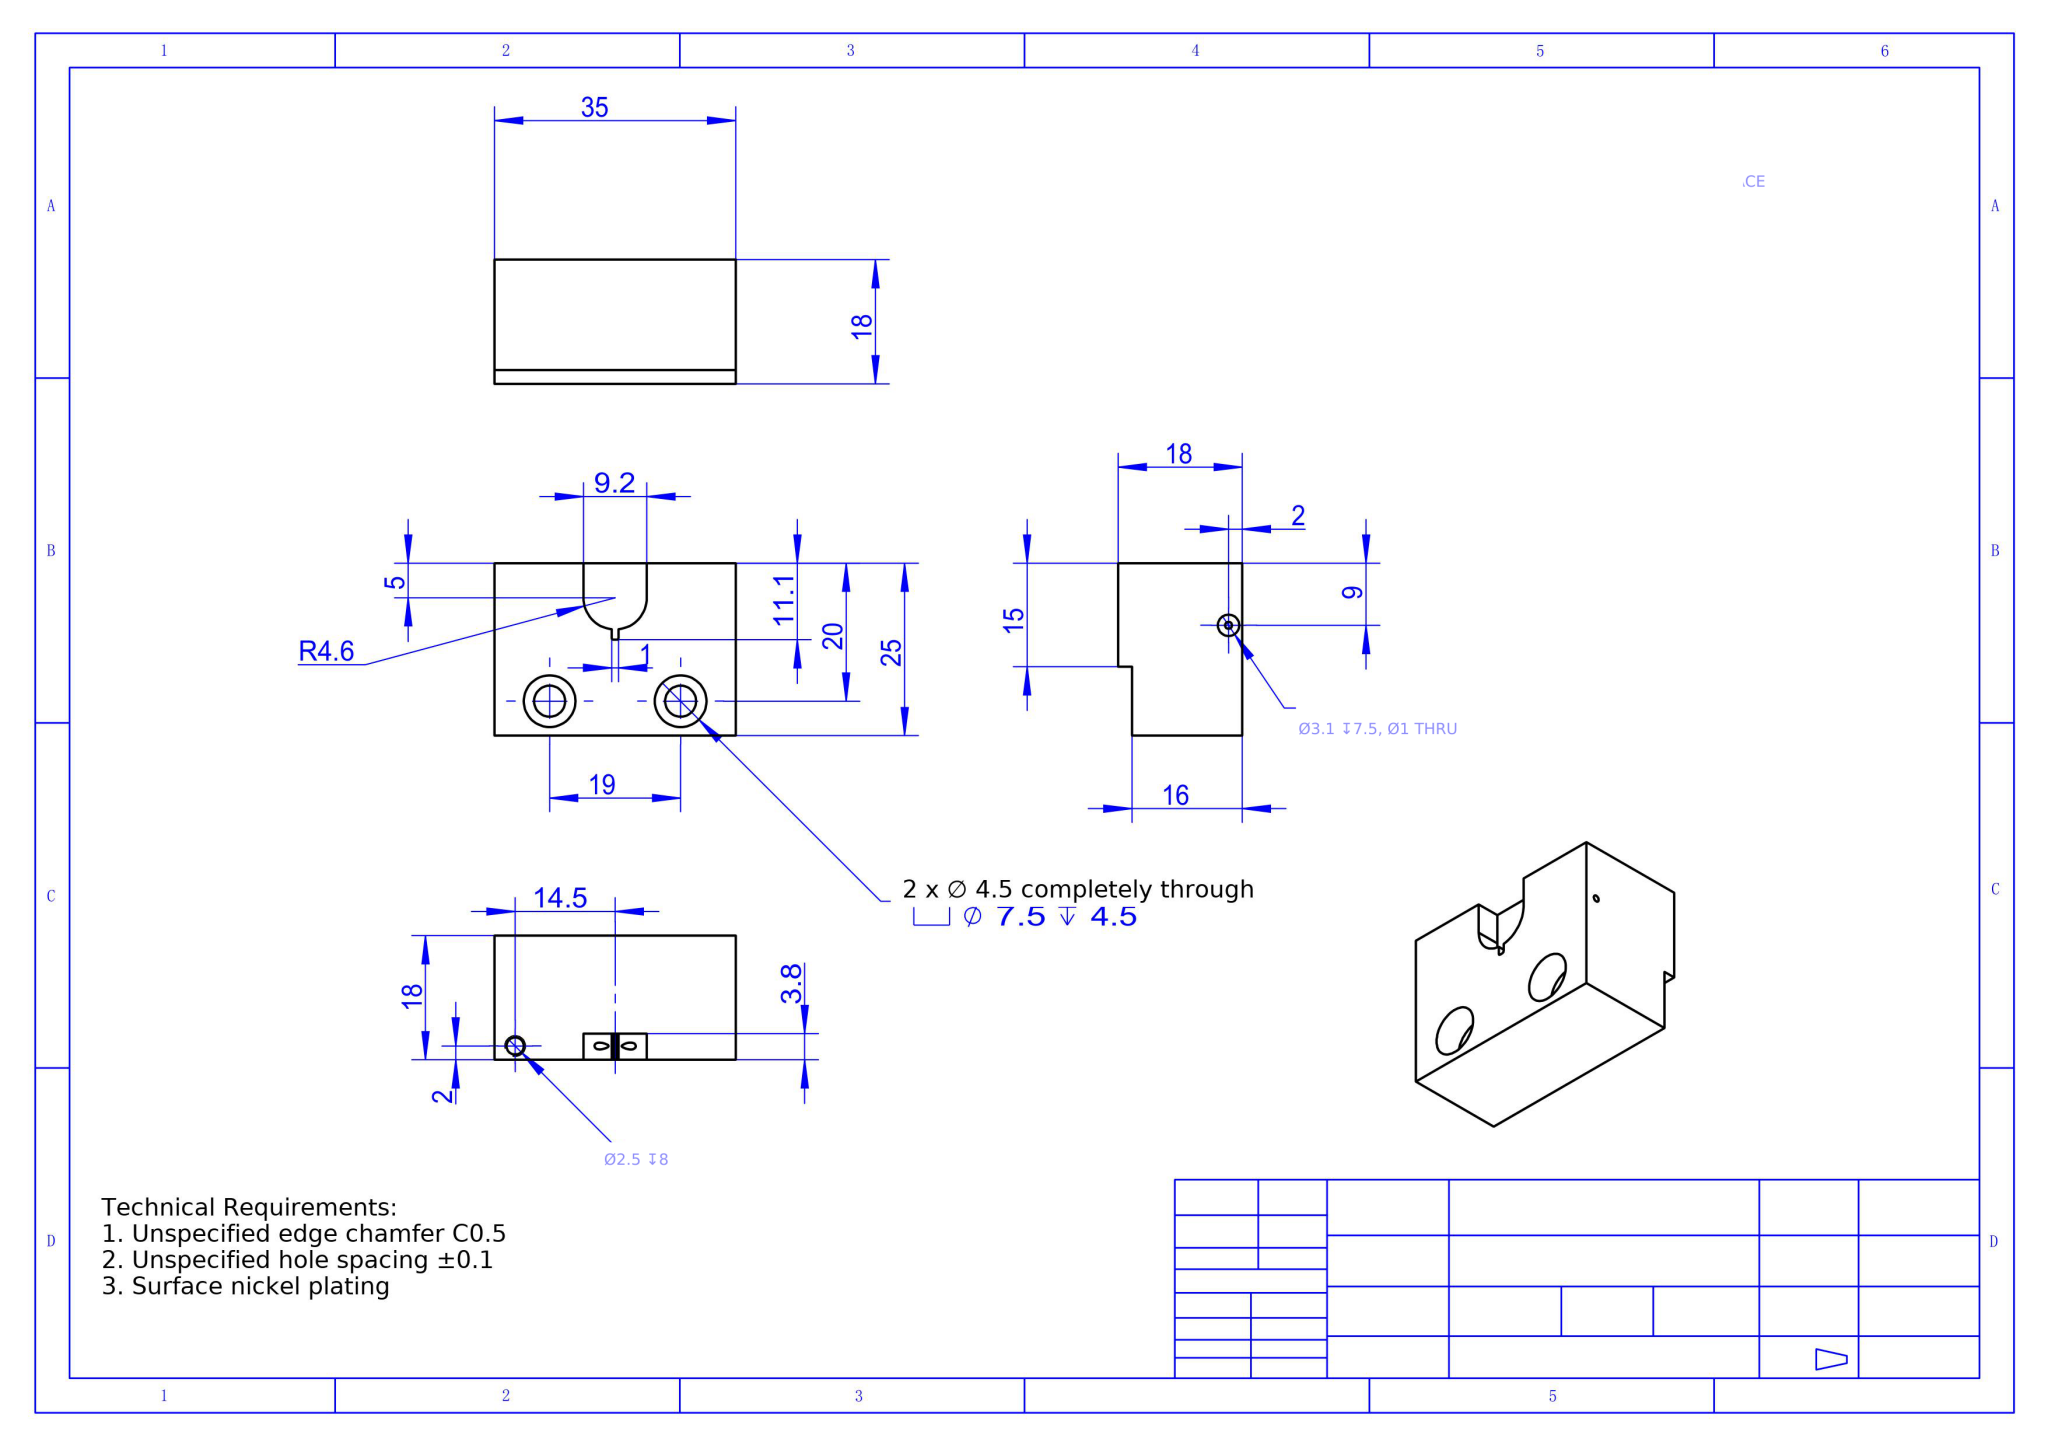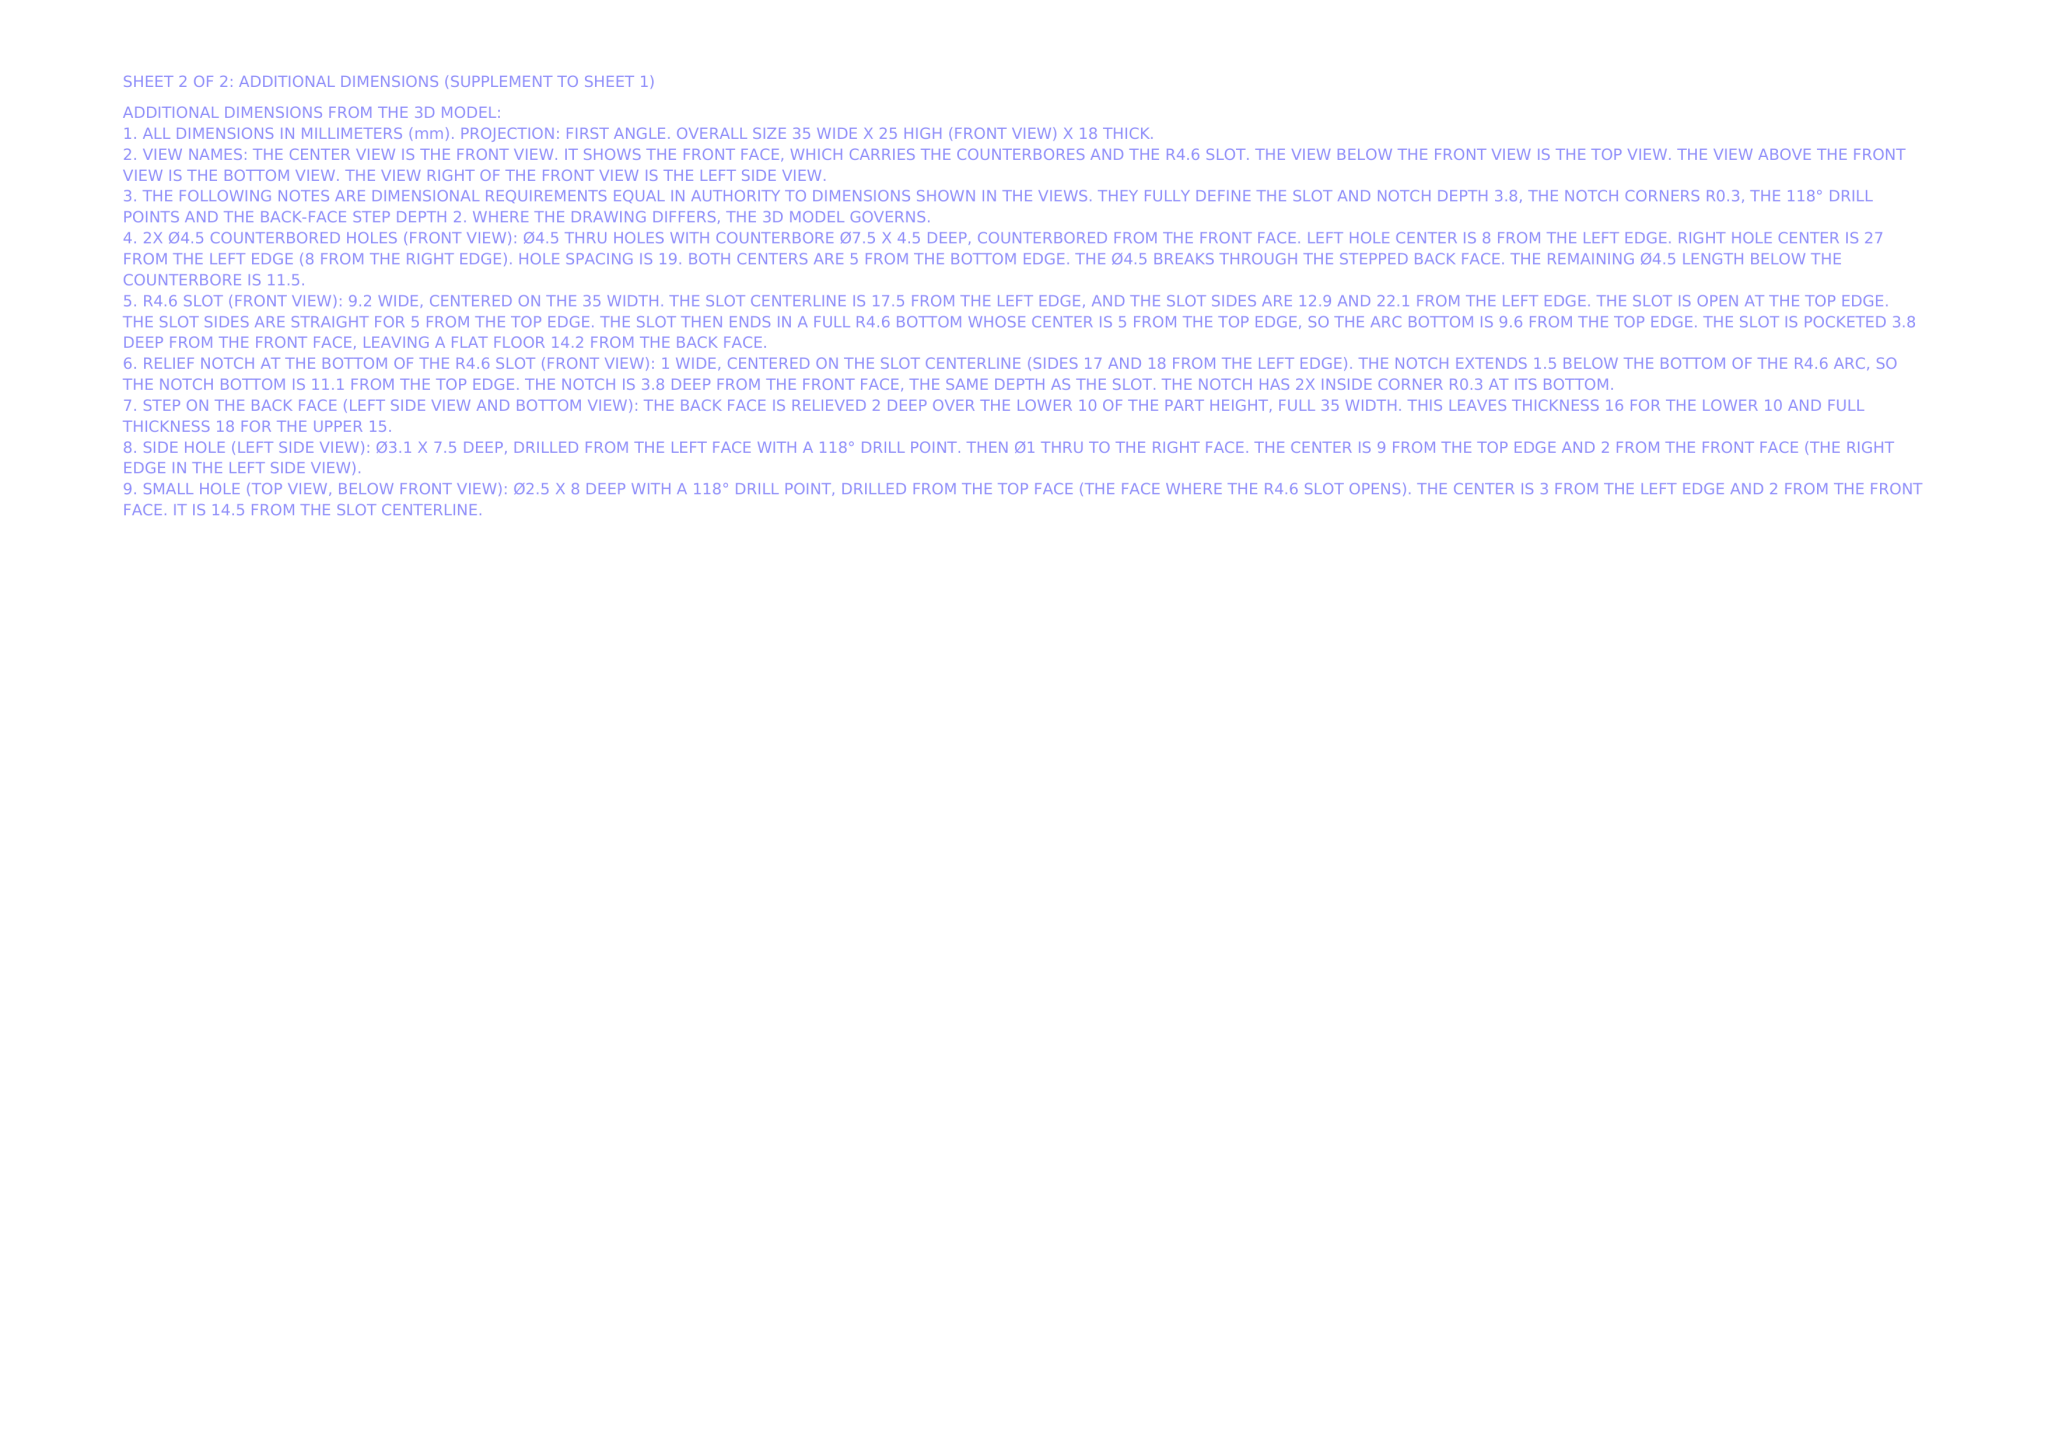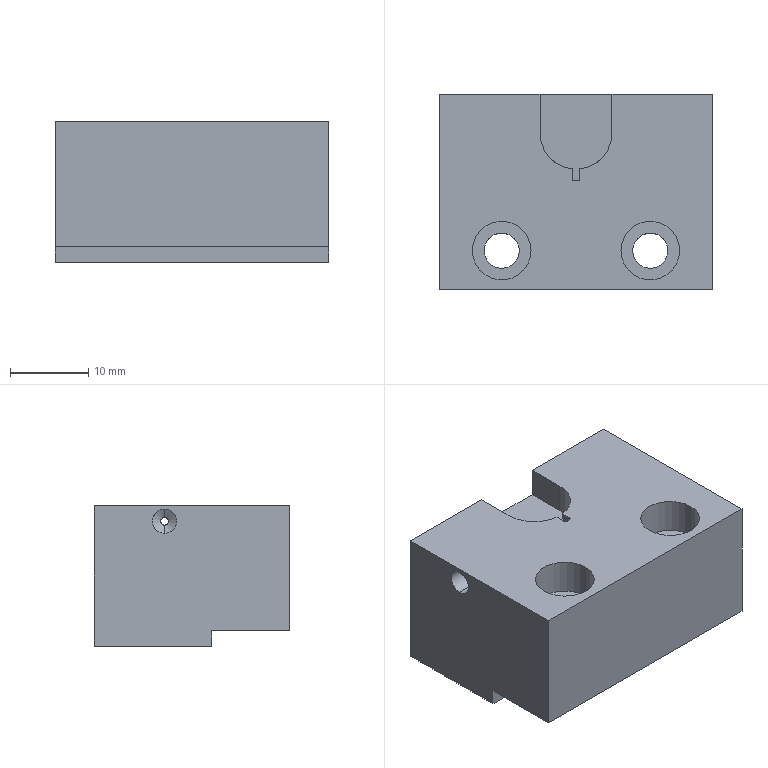Part | NX | mm | 1 solid | 41 faces | box 35 x 25 x 18 mm | volume 13866 mm3 | cylinder 20 | plane 16 | cone 5 | commonest cylinder face diameters 1 x4 7.5 x4 4.5 x4 2.5 x2 3.1 x2 9.2 x2 0.6 x2